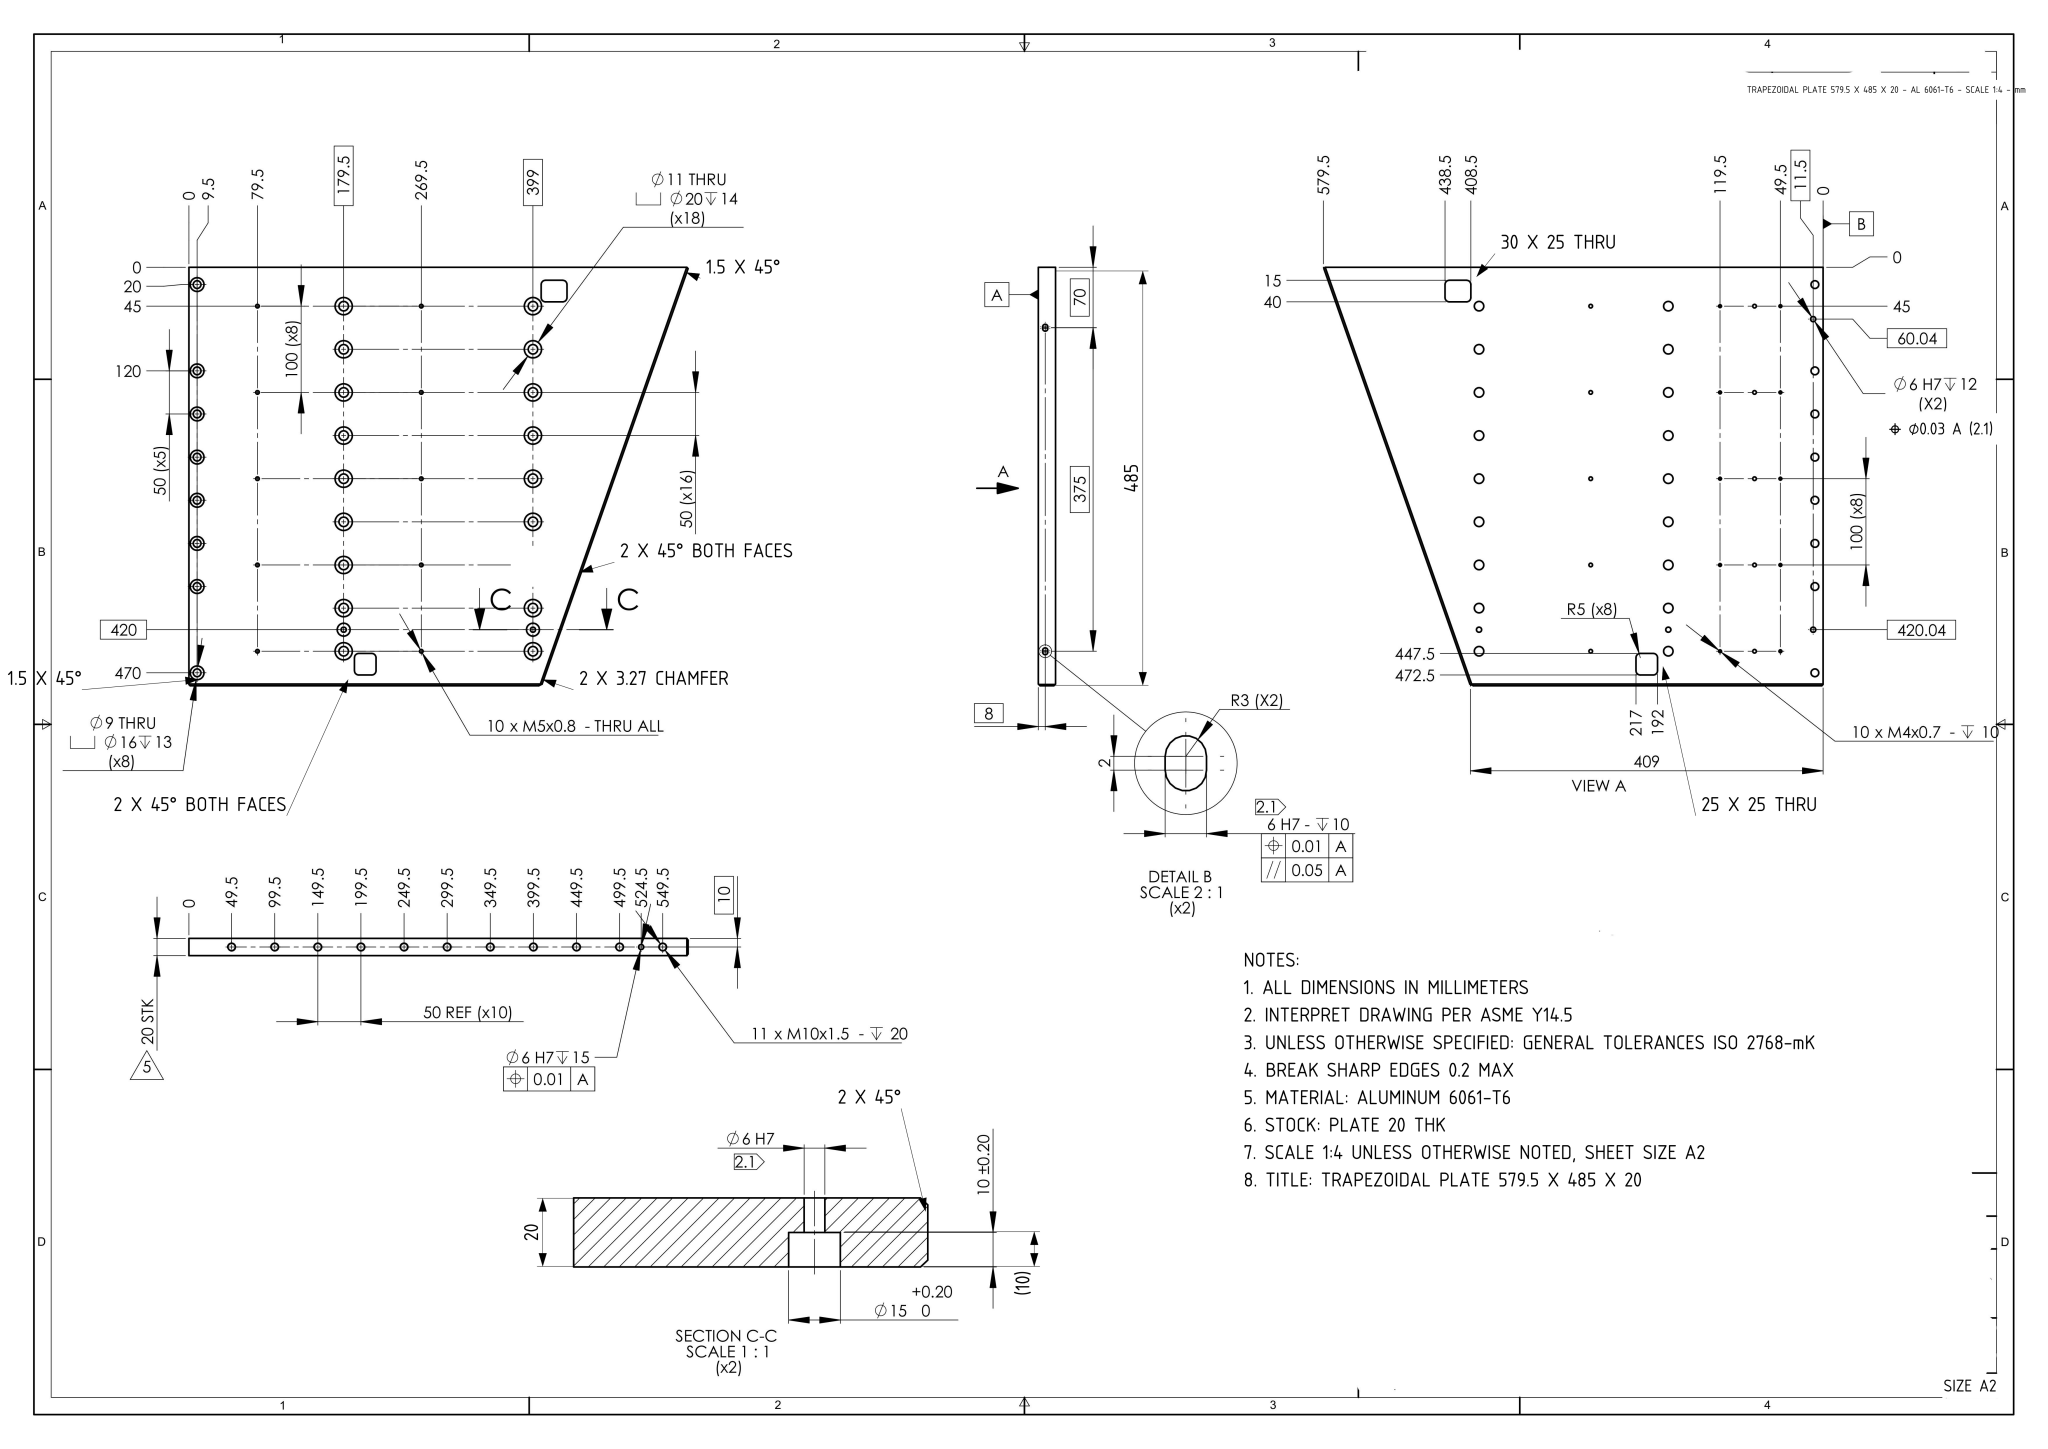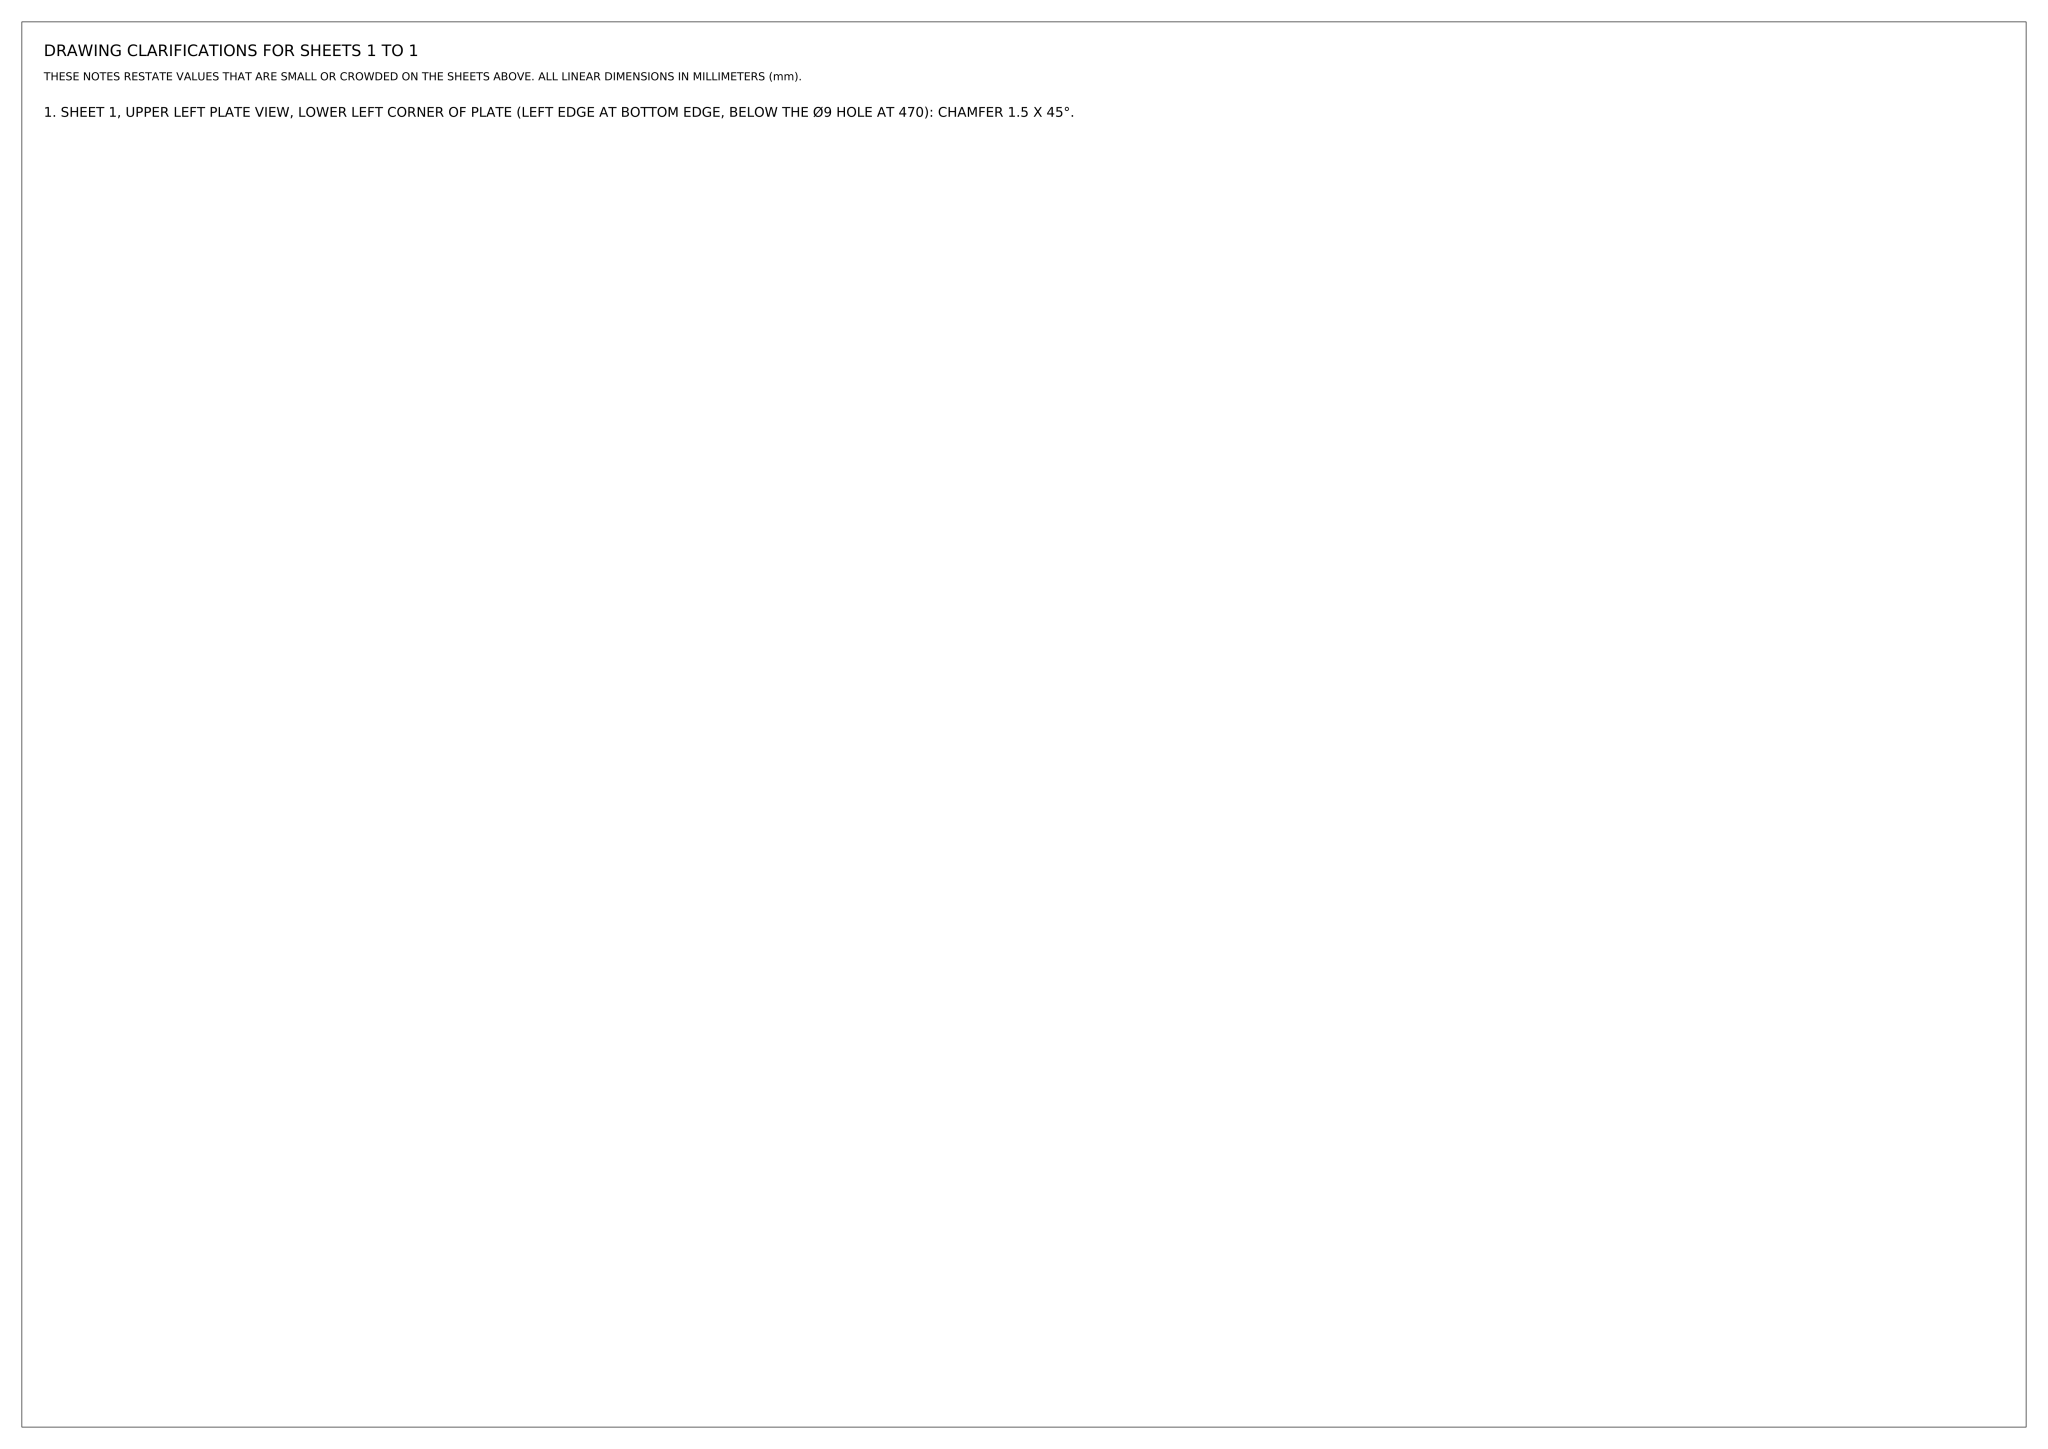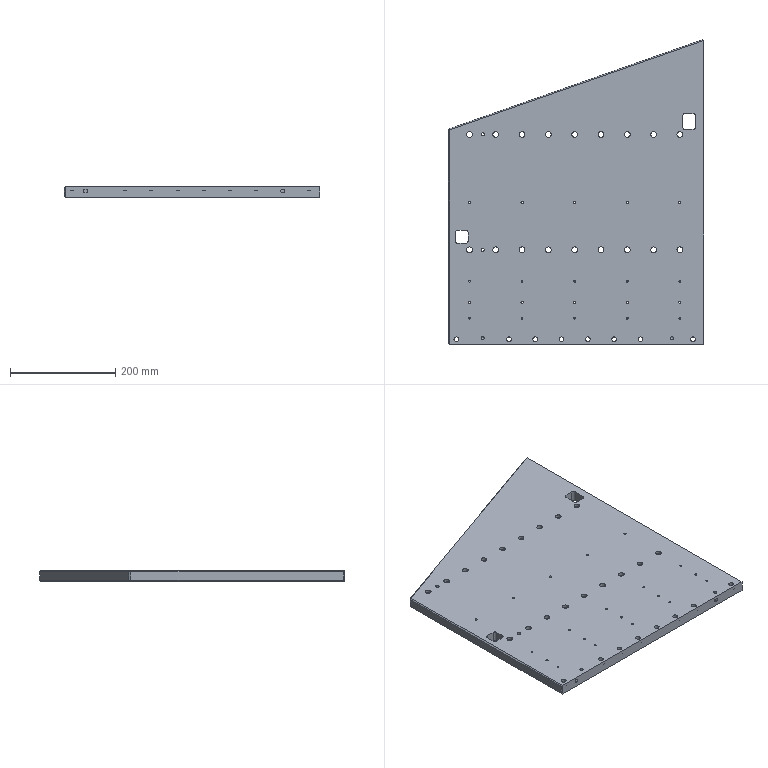Part | NX | mm | 1 solid | 297 faces | box 485 x 578.98 x 20 mm | volume 4624216 mm3 | cylinder 192 | plane 57 | cone 48 | commonest cylinder face diameters 11 x36 20 x36 8.5 x22 3.3 x20 4.2 x20 9 x16 16 x16 6 x14